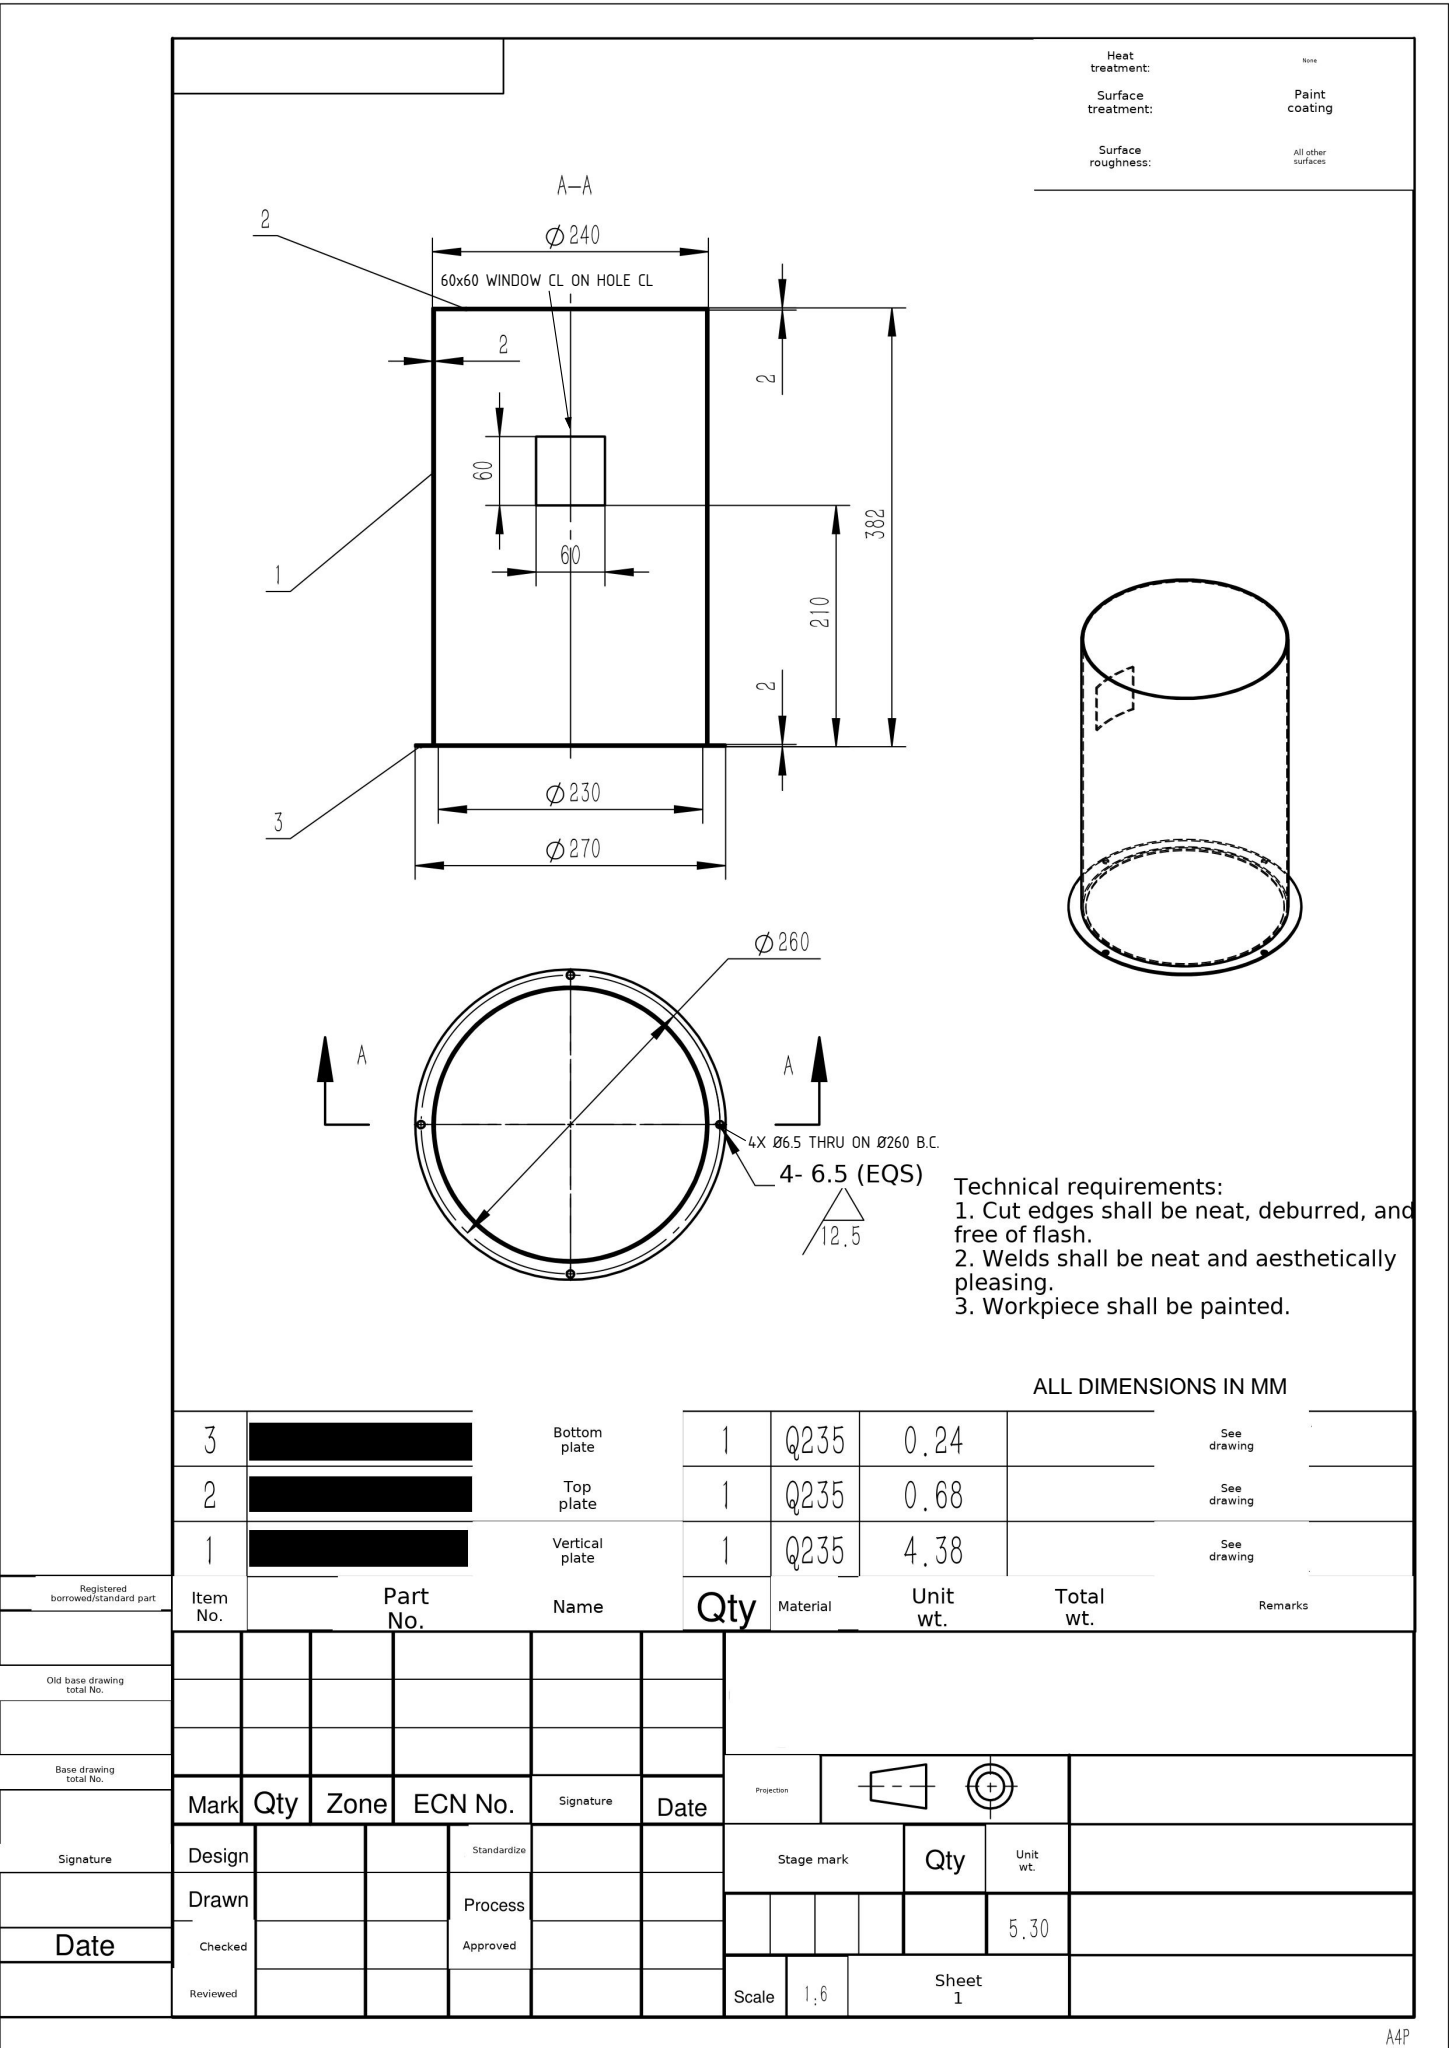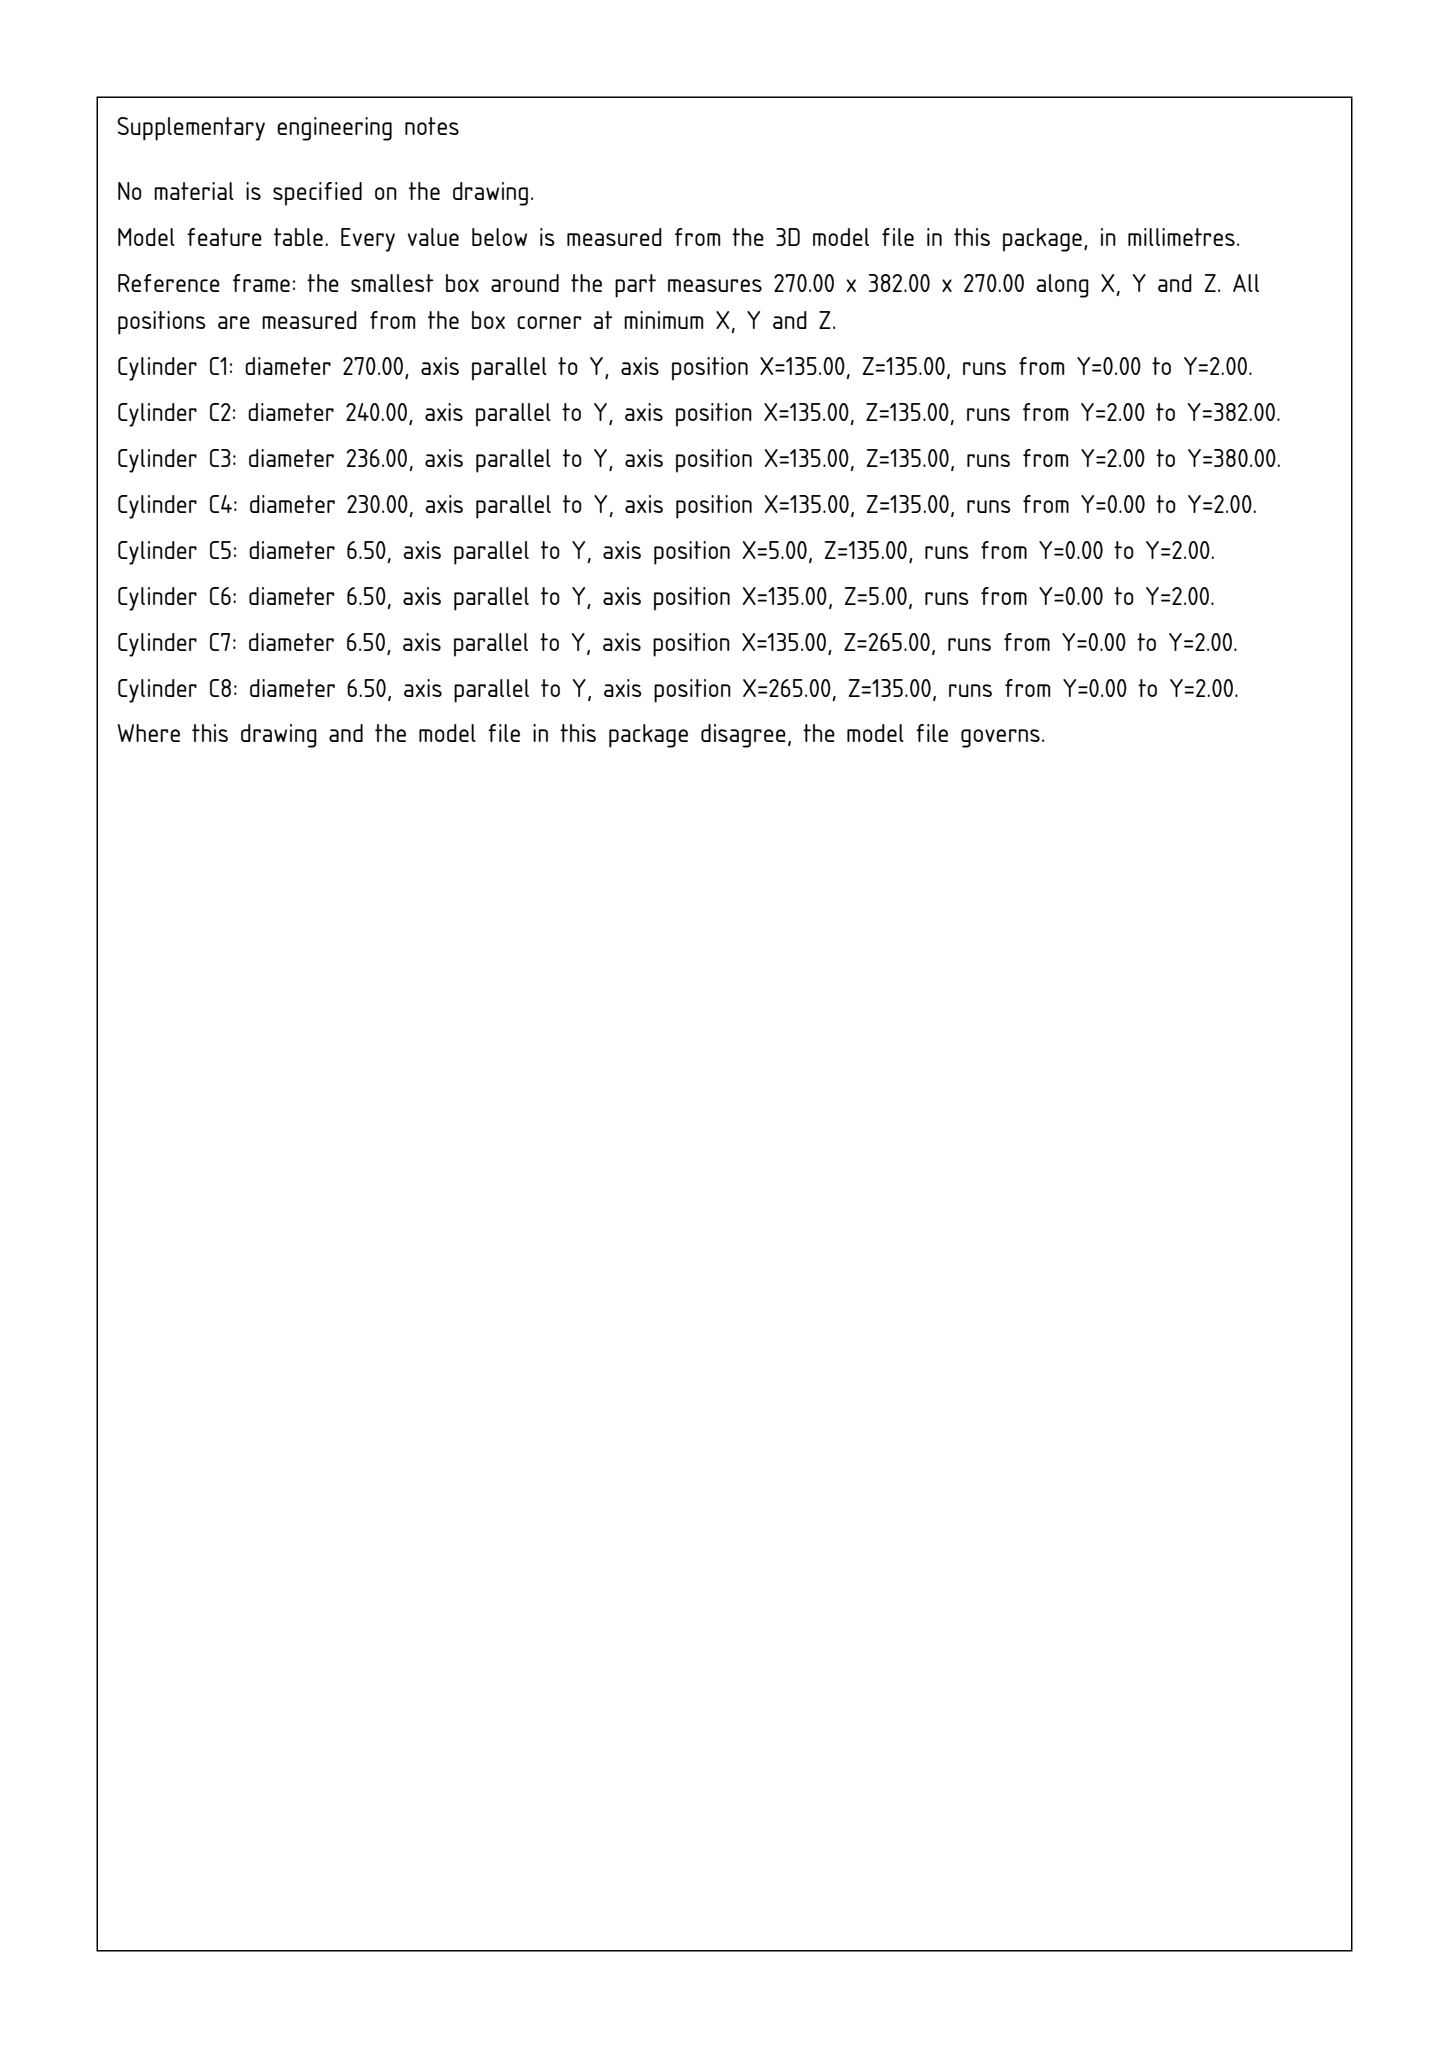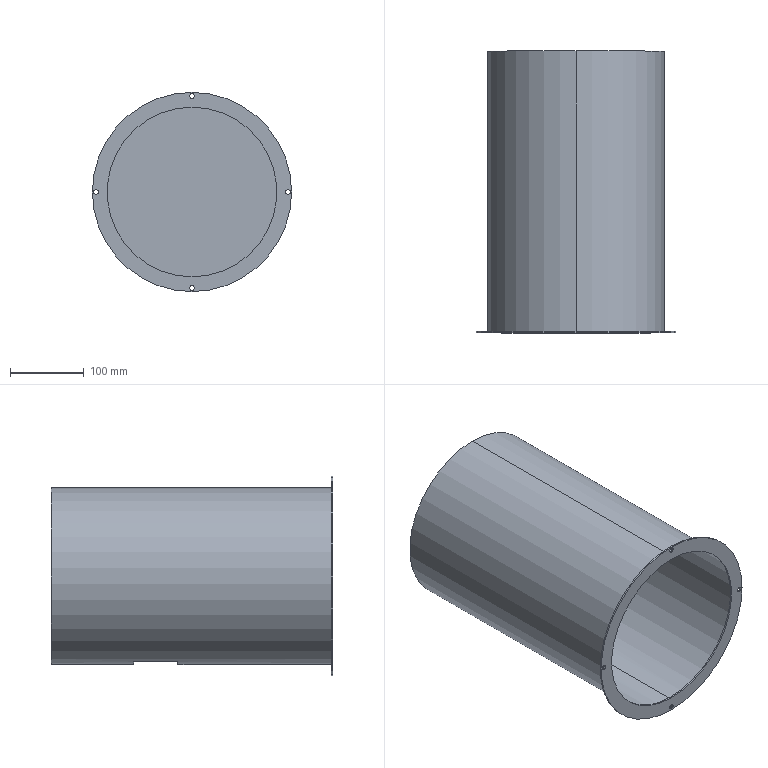Part | SolidWorks | mm | material Q235 | 1 solid | 25 faces | box 270 x 382 x 270 mm | volume 679610 mm3 | cylinder 16 | plane 9 | commonest cylinder face diameters 6.5 x8 230 x2 270 x2 240 x2 236 x2
Drawing notes:
60x60 WINDOW CL ALIGNED W/ ONE 4X Ø6.5 HOLE RADIAL CL (0°) | from the solid: Window faces x=105/165 (CL x=135), z=18.8-20.9; cyl axis at x=135,z=135; Ø6.5 hole at (135,5) lies on same x=135 radial CL
4X Ø6.5 THRU BOTTOM PLATE, EQ SP ON Ø260 B.C. | from the solid: Four Ø6.5 bores, axis y, from y=0 to 2 (2 thk bottom plate), at (135,265),(135,5),(265,135),(5,135) = R130 from axis (135,135)
build123d program:
from build123d import *

# Parameters (mm, degrees)
SKETCH2_R           = 120
SKETCH2_R_2         = 118
BOSS_EXTRUDE1_DEPTH = 380
SKETCH3_R           = 118
BOSS_EXTRUDE2_DEPTH = 2
SKETCH4_R           = 135
SKETCH4_R_2         = 115
BOSS_EXTRUDE3_DEPTH = 2
SKETCH5_R           = 3.25
CUT_EXTRUDE1_DEPTH  = 10
CIRPATTERN1_COUNT   = 4
SKETCH7_W           = 60
SKETCH7_H           = 60
CUT_EXTRUDE5_DEPTH  = 426.265


with BuildPart() as part:
    # Sketch2 → Boss-Extrude1 (new body)
    with BuildSketch(Plane(origin=(0, 0, 0), x_dir=(1, 0, 0), z_dir=(0, 1, 0))):
        with Locations(Location((0, 0, 0), (0, 0, 270))):
            Circle(SKETCH2_R)
        with Locations(Location((0, 0, 0), (0, 0, 270))):
            Circle(SKETCH2_R_2, mode=Mode.SUBTRACT)
    extrude(amount=BOSS_EXTRUDE1_DEPTH)

    # Sketch7 → Cut-Extrude5 (cut, through all)
    with BuildSketch(Plane.XY):
        with Locations((0, 238)):
            Rectangle(SKETCH7_W, SKETCH7_H)
    extrude(amount=-CUT_EXTRUDE5_DEPTH, mode=Mode.SUBTRACT)


with BuildPart() as body_2:
    # Sketch3 → Boss-Extrude2 (new body)
    with BuildSketch(Plane(origin=(0, 380, 0), x_dir=(1, 0, 0), z_dir=(0, 1, 0))):
        with Locations(Location((0, 0, 0), (0, 0, 270))):
            Circle(SKETCH3_R)
    extrude(amount=-BOSS_EXTRUDE2_DEPTH)


with BuildPart() as body_3:
    # Sketch4 → Boss-Extrude3 (new body)
    with BuildSketch(Plane.XZ):
        with Locations(Location((0, 0, 0), (0, 0, 270))):
            Circle(SKETCH4_R)
        with Locations(Location((0, 0, 0), (0, 0, 270))):
            Circle(SKETCH4_R_2, mode=Mode.SUBTRACT)
    extrude(amount=BOSS_EXTRUDE3_DEPTH)

    # Sketch5 → Cut-Extrude1 (cut)
    with BuildSketch(Plane(origin=(0, 0, 0), x_dir=(1, 0, 0), z_dir=(0, 1, 0))):
        with Locations(Location((0, 130, 0), (0, 0, 270))):
            Circle(SKETCH5_R)
    cut_extrude1 = extrude(amount=-CUT_EXTRUDE1_DEPTH, mode=Mode.SUBTRACT)

    # CirPattern1: Cut-Extrude1 ×4 about axis
    cirpattern1_axis = Axis((0, 0, 0), (0, 1, 0))
    for i in range(1, CIRPATTERN1_COUNT):
        add(cut_extrude1.rotate(cirpattern1_axis, i * 360 / CIRPATTERN1_COUNT), mode=Mode.SUBTRACT)


with BuildPart() as part_1:
    add(part.part)

    # Combine-RayDong-Repair: union body 2, body 3
    add(body_2.part)
    add(body_3.part)


solid = part_1.part
STEP:
#1=CARTESIAN_POINT('',(0.,-2.,126.75));
#2=VERTEX_POINT('',#1);
#3=CARTESIAN_POINT('',(-0.,-2.,133.25));
#4=VERTEX_POINT('',#3);
#5=CARTESIAN_POINT('',(0.,-2.,130.));
#6=DIRECTION('',(0.,-1.,0.));
#7=DIRECTION('',(0.,0.,1.));
#8=AXIS2_PLACEMENT_3D('',#5,#6,#7);
#9=CIRCLE('',#8,3.25);
#10=EDGE_CURVE('',#2,#4,#9,.T.);
#11=ORIENTED_EDGE('',*,*,#10,.T.);
#12=CARTESIAN_POINT('',(-0.,0.,133.25));
#13=VERTEX_POINT('',#12);
#14=CARTESIAN_POINT('',(-0.,-10.,133.25));
#15=DIRECTION('',(0.,1.,0.));
#16=VECTOR('',#15,1000.);
#17=LINE('',#14,#16);
#18=EDGE_CURVE('',#4,#13,#17,.T.);
#19=ORIENTED_EDGE('',*,*,#18,.T.);
#20=CARTESIAN_POINT('',(0.,0.,126.75));
#21=VERTEX_POINT('',#20);
#22=CARTESIAN_POINT('',(0.,0.,130.));
#23=DIRECTION('',(0.,1.,0.));
#24=DIRECTION('',(0.,0.,-1.));
#25=AXIS2_PLACEMENT_3D('',#22,#23,#24);
#26=CIRCLE('',#25,3.25);
#27=EDGE_CURVE('',#13,#21,#26,.T.);
#28=ORIENTED_EDGE('',*,*,#27,.T.);
#29=CARTESIAN_POINT('',(0.,-10.,126.75));
#30=DIRECTION('',(0.,1.,0.));
#31=VECTOR('',#30,1000.);
#32=LINE('',#29,#31);
#33=EDGE_CURVE('',#2,#21,#32,.T.);
#34=ORIENTED_EDGE('',*,*,#33,.F.);
#35=EDGE_LOOP('',(#11,#19,#28,#34));
#36=FACE_OUTER_BOUND('',#35,.T.);
#37=CARTESIAN_POINT('',(0.,-10.,130.));
#38=DIRECTION('',(0.,1.,0.));
#39=DIRECTION('',(0.,0.,-1.));
#40=AXIS2_PLACEMENT_3D('',#37,#38,#39);
#41=CYLINDRICAL_SURFACE('',#40,3.25);
#42=ADVANCED_FACE('',(#36),#41,.F.);
#43=CARTESIAN_POINT('',(126.75,-2.,-0.));
#44=VERTEX_POINT('',#43);
#45=CARTESIAN_POINT('',(133.25,-2.,-0.));
#46=VERTEX_POINT('',#45);
#47=CARTESIAN_POINT('',(130.,-2.,-0.));
#48=DIRECTION('',(0.,-1.,0.));
#49=DIRECTION('',(1.,0.,-0.));
#50=AXIS2_PLACEMENT_3D('',#47,#48,#49);
#51=CIRCLE('',#50,3.25);
#52=EDGE_CURVE('',#44,#46,#51,.T.);
#53=ORIENTED_EDGE('',*,*,#52,.T.);
#54=CARTESIAN_POINT('',(133.25,0.,-0.));
#55=VERTEX_POINT('',#54);
#56=CARTESIAN_POINT('',(133.25,-10.,-0.));
#57=DIRECTION('',(0.,1.,0.));
#58=VECTOR('',#57,1000.);
#59=LINE('',#56,#58);
#60=EDGE_CURVE('',#46,#55,#59,.T.);
#61=ORIENTED_EDGE('',*,*,#60,.T.);
#62=CARTESIAN_POINT('',(126.75,0.,-0.));
#63=VERTEX_POINT('',#62);
#64=CARTESIAN_POINT('',(130.,0.,-0.));
#65=DIRECTION('',(0.,1.,0.));
#66=DIRECTION('',(-1.,0.,0.));
#67=AXIS2_PLACEMENT_3D('',#64,#65,#66);
#68=CIRCLE('',#67,3.25);
#69=EDGE_CURVE('',#55,#63,#68,.T.);
#70=ORIENTED_EDGE('',*,*,#69,.T.);
#71=CARTESIAN_POINT('',(126.75,-10.,-0.));
#72=DIRECTION('',(0.,1.,0.));
#73=VECTOR('',#72,1000.);
#74=LINE('',#71,#73);
#75=EDGE_CURVE('',#44,#63,#74,.T.);
#76=ORIENTED_EDGE('',*,*,#75,.F.);
#77=EDGE_LOOP('',(#53,#61,#70,#76));
#78=FACE_OUTER_BOUND('',#77,.T.);
#79=CARTESIAN_POINT('',(130.,-10.,-0.));
#80=DIRECTION('',(0.,1.,0.));
#81=DIRECTION('',(-1.,0.,0.));
#82=AXIS2_PLACEMENT_3D('',#79,#80,#81);
#83=CYLINDRICAL_SURFACE('',#82,3.25);
#84=ADVANCED_FACE('',(#78),#83,.F.);
#85=CARTESIAN_POINT('',(-126.75,-2.,0.));
#86=VERTEX_POINT('',#85);
#87=CARTESIAN_POINT('',(-133.25,-2.,0.));
#88=VERTEX_POINT('',#87);
#89=CARTESIAN_POINT('',(-130.,-2.,0.));
#90=DIRECTION('',(0.,-1.,0.));
#91=DIRECTION('',(-1.,0.,0.));
#92=AXIS2_PLACEMENT_3D('',#89,#90,#91);
#93=CIRCLE('',#92,3.25);
#94=EDGE_CURVE('',#86,#88,#93,.T.);
#95=ORIENTED_EDGE('',*,*,#94,.T.);
#96=CARTESIAN_POINT('',(-133.25,0.,0.));
#97=VERTEX_POINT('',#96);
#98=CARTESIAN_POINT('',(-133.25,-10.,0.));
#99=DIRECTION('',(0.,1.,0.));
#100=VECTOR('',#99,1000.);
#101=LINE('',#98,#100);
#102=EDGE_CURVE('',#88,#97,#101,.T.);
#103=ORIENTED_EDGE('',*,*,#102,.T.);
#104=CARTESIAN_POINT('',(-126.75,0.,0.));
#105=VERTEX_POINT('',#104);
#106=CARTESIAN_POINT('',(-130.,0.,0.));
#107=DIRECTION('',(0.,1.,0.));
#108=DIRECTION('',(1.,0.,-0.));
#109=AXIS2_PLACEMENT_3D('',#106,#107,#108);
#110=CIRCLE('',#109,3.25);
#111=EDGE_CURVE('',#97,#105,#110,.T.);
#112=ORIENTED_EDGE('',*,*,#111,.T.);
#113=CARTESIAN_POINT('',(-126.75,-10.,0.));
#114=DIRECTION('',(0.,1.,0.));
#115=VECTOR('',#114,1000.);
#116=LINE('',#113,#115);
#117=EDGE_CURVE('',#86,#105,#116,.T.);
#118=ORIENTED_EDGE('',*,*,#117,.F.);
#119=EDGE_LOOP('',(#95,#103,#112,#118));
#120=FACE_OUTER_BOUND('',#119,.T.);
#121=CARTESIAN_POINT('',(-130.,-10.,0.));
#122=DIRECTION('',(0.,1.,0.));
#123=DIRECTION('',(1.,0.,-0.));
#124=AXIS2_PLACEMENT_3D('',#121,#122,#123);
#125=CYLINDRICAL_SURFACE('',#124,3.25);
#126=ADVANCED_FACE('',(#120),#125,.F.);
#127=CARTESIAN_POINT('',(0.,-2.,-126.75));
#128=VERTEX_POINT('',#127);
#129=CARTESIAN_POINT('',(0.,-2.,-133.25));
#130=VERTEX_POINT('',#129);
#131=CARTESIAN_POINT('',(0.,-2.,-130.));
#132=DIRECTION('',(0.,-1.,0.));
#133=DIRECTION('',(0.,0.,-1.));
#134=AXIS2_PLACEMENT_3D('',#131,#132,#133);
#135=CIRCLE('',#134,3.25);
#136=EDGE_CURVE('',#128,#130,#135,.T.);
#137=ORIENTED_EDGE('',*,*,#136,.T.);
#138=CARTESIAN_POINT('',(0.,0.,-133.25));
#139=VERTEX_POINT('',#138);
#140=CARTESIAN_POINT('',(0.,-10.,-133.25));
#141=DIRECTION('',(0.,1.,0.));
#142=VECTOR('',#141,1000.);
#143=LINE('',#140,#142);
#144=EDGE_CURVE('',#130,#139,#143,.T.);
#145=ORIENTED_EDGE('',*,*,#144,.T.);
#146=CARTESIAN_POINT('',(0.,0.,-126.75));
#147=VERTEX_POINT('',#146);
#148=CARTESIAN_POINT('',(0.,0.,-130.));
#149=DIRECTION('',(0.,1.,0.));
#150=DIRECTION('',(0.,0.,1.));
#151=AXIS2_PLACEMENT_3D('',#148,#149,#150);
#152=CIRCLE('',#151,3.25);
#153=EDGE_CURVE('',#139,#147,#152,.T.);
#154=ORIENTED_EDGE('',*,*,#153,.T.);
#155=CARTESIAN_POINT('',(0.,-10.,-126.75));
#156=DIRECTION('',(0.,1.,0.));
#157=VECTOR('',#156,1000.);
#158=LINE('',#155,#157);
#159=EDGE_CURVE('',#128,#147,#158,.T.);
#160=ORIENTED_EDGE('',*,*,#159,.F.);
#161=EDGE_LOOP('',(#137,#145,#154,#160));
#162=FACE_OUTER_BOUND('',#161,.T.);
#163=CARTESIAN_POINT('',(0.,-10.,-130.));
#164=DIRECTION('',(0.,1.,0.));
#165=DIRECTION('',(0.,0.,1.));
#166=AXIS2_PLACEMENT_3D('',#163,#164,#165);
#167=CYLINDRICAL_SURFACE('',#166,3.25);
#168=ADVANCED_FACE('',(#162),#167,.F.);
#169=CARTESIAN_POINT('',(0.,-2.,115.));
#170=VERTEX_POINT('',#169);
#171=CARTESIAN_POINT('',(0.,-2.,-115.));
#172=VERTEX_POINT('',#171);
#173=CARTESIAN_POINT('',(0.,-2.,0.));
#174=DIRECTION('',(0.,-1.,0.));
#175=DIRECTION('',(0.,0.,-1.));
#176=AXIS2_PLACEMENT_3D('',#173,#174,#175);
#177=CIRCLE('',#176,115.);
#178=EDGE_CURVE('',#170,#172,#177,.T.);
#179=ORIENTED_EDGE('',*,*,#178,.T.);
#180=CARTESIAN_POINT('',(0.,0.,-115.));
#181=VERTEX_POINT('',#180);
#182=CARTESIAN_POINT('',(0.,-2.,-115.));
#183=DIRECTION('',(0.,1.,0.));
#184=VECTOR('',#183,1000.);
#185=LINE('',#182,#184);
#186=EDGE_CURVE('',#172,#181,#185,.T.);
#187=ORIENTED_EDGE('',*,*,#186,.T.);
#188=CARTESIAN_POINT('',(0.,0.,115.));
#189=VERTEX_POINT('',#188);
#190=CARTESIAN_POINT('',(0.,0.,0.));
#191=DIRECTION('',(0.,-1.,0.));
#192=DIRECTION('',(0.,0.,-1.));
#193=AXIS2_PLACEMENT_3D('',#190,#191,#192);
#194=CIRCLE('',#193,115.);
#195=EDGE_CURVE('',#189,#181,#194,.T.);
#196=ORIENTED_EDGE('',*,*,#195,.F.);
#197=CARTESIAN_POINT('',(0.,-2.,115.));
#198=DIRECTION('',(0.,1.,0.));
#199=VECTOR('',#198,1000.);
#200=LINE('',#197,#199);
#201=EDGE_CURVE('',#170,#189,#200,.T.);
#202=ORIENTED_EDGE('',*,*,#201,.F.);
#203=EDGE_LOOP('',(#179,#187,#196,#202));
#204=FACE_OUTER_BOUND('',#203,.T.);
#205=CARTESIAN_POINT('',(0.,-2.,0.));
#206=DIRECTION('',(0.,1.,0.));
#207=DIRECTION('',(0.,0.,1.));
#208=AXIS2_PLACEMENT_3D('',#205,#206,#207);
#209=CYLINDRICAL_SURFACE('',#208,115.);
#210=ADVANCED_FACE('',(#204),#209,.F.);
#211=CARTESIAN_POINT('',(0.,-2.,-135.));
#212=VERTEX_POINT('',#211);
#213=CARTESIAN_POINT('',(0.,-2.,135.));
#214=VERTEX_POINT('',#213);
#215=CARTESIAN_POINT('',(0.,-2.,0.));
#216=DIRECTION('',(0.,-1.,0.));
#217=DIRECTION('',(0.,0.,-1.));
#218=AXIS2_PLACEMENT_3D('',#215,#216,#217);
#219=CIRCLE('',#218,135.);
#220=EDGE_CURVE('',#212,#214,#219,.T.);
#221=ORIENTED_EDGE('',*,*,#220,.F.);
#222=CARTESIAN_POINT('',(0.,0.,-135.));
#223=VERTEX_POINT('',#222);
#224=CARTESIAN_POINT('',(0.,-2.,-135.));
#225=DIRECTION('',(0.,1.,0.));
#226=VECTOR('',#225,1000.);
#227=LINE('',#224,#226);
#228=EDGE_CURVE('',#212,#223,#227,.T.);
#229=ORIENTED_EDGE('',*,*,#228,.T.);
#230=CARTESIAN_POINT('',(0.,0.,135.));
#231=VERTEX_POINT('',#230);
#232=CARTESIAN_POINT('',(0.,0.,0.));
#233=DIRECTION('',(0.,-1.,0.));
#234=DIRECTION('',(0.,0.,-1.));
#235=AXIS2_PLACEMENT_3D('',#232,#233,#234);
#236=CIRCLE('',#235,135.);
#237=EDGE_CURVE('',#223,#231,#236,.T.);
#238=ORIENTED_EDGE('',*,*,#237,.T.);
#239=CARTESIAN_POINT('',(0.,-2.,135.));
#240=DIRECTION('',(0.,1.,0.));
#241=VECTOR('',#240,1000.);
#242=LINE('',#239,#241);
#243=EDGE_CURVE('',#214,#231,#242,.T.);
#244=ORIENTED_EDGE('',*,*,#243,.F.);
#245=EDGE_LOOP('',(#221,#229,#238,#244));
#246=FACE_OUTER_BOUND('',#245,.T.);
#247=CARTESIAN_POINT('',(0.,-2.,0.));
#248=DIRECTION('',(0.,1.,0.));
#249=DIRECTION('',(0.,0.,1.));
#250=AXIS2_PLACEMENT_3D('',#247,#248,#249);
#251=CYLINDRICAL_SURFACE('',#250,135.);
#252=ADVANCED_FACE('',(#246),#251,.T.);
#253=CARTESIAN_POINT('',(0.,380.,120.));
#254=VERTEX_POINT('',#253);
#255=CARTESIAN_POINT('',(0.,380.,-120.));
#256=VERTEX_POINT('',#255);
#257=CARTESIAN_POINT('',(0.,380.,0.));
#258=DIRECTION('',(0.,1.,0.));
#259=DIRECTION('',(0.,0.,1.));
#260=AXIS2_PLACEMENT_3D('',#257,#258,#259);
#261=CIRCLE('',#260,120.);
#262=EDGE_CURVE('',#254,#256,#261,.T.);
#263=ORIENTED_EDGE('',*,*,#262,.F.);
#264=CARTESIAN_POINT('',(0.,0.,120.));
#265=VERTEX_POINT('',#264);
#266=CARTESIAN_POINT('',(0.,380.,120.));
#267=DIRECTION('',(0.,-1.,0.));
#268=VECTOR('',#267,1000.);
#269=LINE('',#266,#268);
#270=EDGE_CURVE('',#254,#265,#269,.T.);
#271=ORIENTED_EDGE('',*,*,#270,.T.);
#272=CARTESIAN_POINT('',(0.,0.,-120.));
#273=VERTEX_POINT('',#272);
#274=CARTESIAN_POINT('',(0.,0.,0.));
#275=DIRECTION('',(0.,1.,0.));
#276=DIRECTION('',(0.,0.,1.));
#277=AXIS2_PLACEMENT_3D('',#274,#275,#276);
#278=CIRCLE('',#277,120.);
#279=EDGE_CURVE('',#265,#273,#278,.T.);
#280=ORIENTED_EDGE('',*,*,#279,.T.);
#281=CARTESIAN_POINT('',(0.,208.,-120.));
#282=VERTEX_POINT('',#281);
#283=CARTESIAN_POINT('',(0.,380.,-120.));
#284=DIRECTION('',(0.,-1.,0.));
#285=VECTOR('',#284,1000.);
#286=LINE('',#283,#285);
#287=EDGE_CURVE('',#282,#273,#286,.T.);
#288=ORIENTED_EDGE('',*,*,#287,.F.);
#289=CARTESIAN_POINT('',(30.,208.,-116.19));
#290=VERTEX_POINT('',#289);
#291=CARTESIAN_POINT('',(0.,208.,0.));
#292=DIRECTION('',(0.,-1.,0.));
#293=DIRECTION('',(0.,0.,-1.));
#294=AXIS2_PLACEMENT_3D('',#291,#292,#293);
#295=CIRCLE('',#294,120.);
#296=EDGE_CURVE('',#282,#290,#295,.T.);
#297=ORIENTED_EDGE('',*,*,#296,.T.);
#298=CARTESIAN_POINT('',(30.,268.,-116.19));
#299=VERTEX_POINT('',#298);
#300=CARTESIAN_POINT('',(30.,380.,-116.19));
#301=DIRECTION('',(0.,1.,0.));
#302=VECTOR('',#301,1000.);
#303=LINE('',#300,#302);
#304=EDGE_CURVE('',#290,#299,#303,.T.);
#305=ORIENTED_EDGE('',*,*,#304,.T.);
#306=CARTESIAN_POINT('',(0.,268.,-120.));
#307=VERTEX_POINT('',#306);
#308=CARTESIAN_POINT('',(0.,268.,0.));
#309=DIRECTION('',(0.,1.,0.));
#310=DIRECTION('',(0.,0.,1.));
#311=AXIS2_PLACEMENT_3D('',#308,#309,#310);
#312=CIRCLE('',#311,120.);
#313=EDGE_CURVE('',#299,#307,#312,.T.);
#314=ORIENTED_EDGE('',*,*,#313,.T.);
#315=CARTESIAN_POINT('',(0.,380.,-120.));
#316=DIRECTION('',(0.,-1.,0.));
#317=VECTOR('',#316,1000.);
#318=LINE('',#315,#317);
#319=EDGE_CURVE('',#256,#307,#318,.T.);
#320=ORIENTED_EDGE('',*,*,#319,.F.);
#321=EDGE_LOOP('',(#263,#271,#280,#288,#297,#305,#314,#320));
#322=FACE_OUTER_BOUND('',#321,.T.);
#323=CARTESIAN_POINT('',(0.,380.,0.));
#324=DIRECTION('',(0.,-1.,0.));
#325=DIRECTION('',(0.,0.,-1.));
#326=AXIS2_PLACEMENT_3D('',#323,#324,#325);
#327=CYLINDRICAL_SURFACE('',#326,120.);
#328=ADVANCED_FACE('',(#322),#327,.T.);
#329=CARTESIAN_POINT('',(0.,378.,-118.));
#330=VERTEX_POINT('',#329);
#331=CARTESIAN_POINT('',(0.,378.,118.));
#332=VERTEX_POINT('',#331);
#333=CARTESIAN_POINT('',(0.,378.,0.));
#334=DIRECTION('',(0.,1.,0.));
#335=DIRECTION('',(0.,0.,1.));
#336=AXIS2_PLACEMENT_3D('',#333,#334,#335);
#337=CIRCLE('',#336,118.);
#338=EDGE_CURVE('',#330,#332,#337,.T.);
#339=ORIENTED_EDGE('',*,*,#338,.T.);
#340=CARTESIAN_POINT('',(0.,0.,118.));
#341=VERTEX_POINT('',#340);
#342=CARTESIAN_POINT('',(0.,380.,118.));
#343=DIRECTION('',(0.,-1.,0.));
#344=VECTOR('',#343,1000.);
#345=LINE('',#342,#344);
#346=EDGE_CURVE('',#332,#341,#345,.T.);
#347=ORIENTED_EDGE('',*,*,#346,.T.);
#348=CARTESIAN_POINT('',(0.,0.,-118.));
#349=VERTEX_POINT('',#348);
#350=CARTESIAN_POINT('',(0.,0.,0.));
#351=DIRECTION('',(0.,1.,0.));
#352=DIRECTION('',(0.,0.,1.));
#353=AXIS2_PLACEMENT_3D('',#350,#351,#352);
#354=CIRCLE('',#353,118.);
#355=EDGE_CURVE('',#349,#341,#354,.T.);
#356=ORIENTED_EDGE('',*,*,#355,.F.);
#357=CARTESIAN_POINT('',(0.,208.,-118.));
#358=VERTEX_POINT('',#357);
#359=CARTESIAN_POINT('',(0.,380.,-118.));
#360=DIRECTION('',(0.,-1.,0.));
#361=VECTOR('',#360,1000.);
#362=LINE('',#359,#361);
#363=EDGE_CURVE('',#358,#349,#362,.T.);
#364=ORIENTED_EDGE('',*,*,#363,.F.);
#365=CARTESIAN_POINT('',(-30.,208.,-114.123));
#366=VERTEX_POINT('',#365);
#367=CARTESIAN_POINT('',(0.,208.,0.));
#368=DIRECTION('',(0.,-1.,0.));
#369=DIRECTION('',(0.,0.,-1.));
#370=AXIS2_PLACEMENT_3D('',#367,#368,#369);
#371=CIRCLE('',#370,118.);
#372=EDGE_CURVE('',#366,#358,#371,.T.);
#373=ORIENTED_EDGE('',*,*,#372,.F.);
#374=CARTESIAN_POINT('',(-30.,268.,-114.123));
#375=VERTEX_POINT('',#374);
#376=CARTESIAN_POINT('',(-30.,380.,-114.123));
#377=DIRECTION('',(0.,-1.,0.));
#378=VECTOR('',#377,1000.);
#379=LINE('',#376,#378);
#380=EDGE_CURVE('',#375,#366,#379,.T.);
#381=ORIENTED_EDGE('',*,*,#380,.F.);
#382=CARTESIAN_POINT('',(0.,268.,-118.));
#383=VERTEX_POINT('',#382);
#384=CARTESIAN_POINT('',(0.,268.,0.));
#385=DIRECTION('',(0.,1.,0.));
#386=DIRECTION('',(0.,0.,1.));
#387=AXIS2_PLACEMENT_3D('',#384,#385,#386);
#388=CIRCLE('',#387,118.);
#389=EDGE_CURVE('',#383,#375,#388,.T.);
#390=ORIENTED_EDGE('',*,*,#389,.F.);
#391=CARTESIAN_POINT('',(0.,380.,-118.));
#392=DIRECTION('',(0.,-1.,0.));
#393=VECTOR('',#392,1000.);
#394=LINE('',#391,#393);
#395=EDGE_CURVE('',#330,#383,#394,.T.);
#396=ORIENTED_EDGE('',*,*,#395,.F.);
#397=EDGE_LOOP('',(#339,#347,#356,#364,#373,#381,#390,#396));
#398=FACE_OUTER_BOUND('',#397,.T.);
#399=CARTESIAN_POINT('',(0.,380.,0.));
#400=DIRECTION('',(0.,-1.,0.));
#401=DIRECTION('',(0.,0.,-1.));
#402=AXIS2_PLACEMENT_3D('',#399,#400,#401);
#403=CYLINDRICAL_SURFACE('',#402,118.);
#404=ADVANCED_FACE('',(#398),#403,.F.);
#405=ORIENTED_EDGE('',*,*,#346,.F.);
#406=CARTESIAN_POINT('',(0.,378.,0.));
#407=DIRECTION('',(0.,1.,0.));
#408=DIRECTION('',(0.,0.,1.));
#409=AXIS2_PLACEMENT_3D('',#406,#407,#408);
#410=CIRCLE('',#409,118.);
#411=EDGE_CURVE('',#332,#330,#410,.T.);
#412=ORIENTED_EDGE('',*,*,#411,.T.);
#413=ORIENTED_EDGE('',*,*,#395,.T.);
#414=CARTESIAN_POINT('',(30.,268.,-114.123));
#415=VERTEX_POINT('',#414);
#416=CARTESIAN_POINT('',(0.,268.,0.));
#417=DIRECTION('',(0.,1.,0.));
#418=DIRECTION('',(0.,0.,1.));
#419=AXIS2_PLACEMENT_3D('',#416,#417,#418);
#420=CIRCLE('',#419,118.);
#421=EDGE_CURVE('',#415,#383,#420,.T.);
#422=ORIENTED_EDGE('',*,*,#421,.F.);
#423=CARTESIAN_POINT('',(30.,208.,-114.123));
#424=VERTEX_POINT('',#423);
#425=CARTESIAN_POINT('',(30.,380.,-114.123));
#426=DIRECTION('',(0.,1.,0.));
#427=VECTOR('',#426,1000.);
#428=LINE('',#425,#427);
#429=EDGE_CURVE('',#424,#415,#428,.T.);
#430=ORIENTED_EDGE('',*,*,#429,.F.);
#431=CARTESIAN_POINT('',(0.,208.,0.));
#432=DIRECTION('',(0.,-1.,0.));
#433=DIRECTION('',(0.,0.,-1.));
#434=AXIS2_PLACEMENT_3D('',#431,#432,#433);
#435=CIRCLE('',#434,118.);
#436=EDGE_CURVE('',#358,#424,#435,.T.);
#437=ORIENTED_EDGE('',*,*,#436,.F.);
#438=ORIENTED_EDGE('',*,*,#363,.T.);
#439=CARTESIAN_POINT('',(0.,0.,0.));
#440=DIRECTION('',(0.,1.,0.));
#441=DIRECTION('',(0.,0.,1.));
#442=AXIS2_PLACEMENT_3D('',#439,#440,#441);
#443=CIRCLE('',#442,118.);
#444=EDGE_CURVE('',#341,#349,#443,.T.);
#445=ORIENTED_EDGE('',*,*,#444,.F.);
#446=EDGE_LOOP('',(#405,#412,#413,#422,#430,#437,#438,#445));
#447=FACE_OUTER_BOUND('',#446,.T.);
#448=CARTESIAN_POINT('',(0.,380.,0.));
#449=DIRECTION('',(0.,-1.,0.));
#450=DIRECTION('',(0.,0.,-1.));
#451=AXIS2_PLACEMENT_3D('',#448,#449,#450);
#452=CYLINDRICAL_SURFACE('',#451,118.);
#453=ADVANCED_FACE('',(#447),#452,.F.);
#454=CARTESIAN_POINT('',(0.,380.,0.));
#455=DIRECTION('',(0.,1.,0.));
#456=DIRECTION('',(0.,0.,1.));
#457=AXIS2_PLACEMENT_3D('',#454,#455,#456);
#458=CIRCLE('',#457,120.);
#459=EDGE_CURVE('',#256,#254,#458,.T.);
#460=ORIENTED_EDGE('',*,*,#459,.T.);
#461=ORIENTED_EDGE('',*,*,#262,.T.);
#462=EDGE_LOOP('',(#460,#461));
#463=FACE_OUTER_BOUND('',#462,.T.);
#464=CARTESIAN_POINT('',(0.,380.,0.));
#465=DIRECTION('',(0.,1.,0.));
#466=DIRECTION('',(0.,0.,1.));
#467=AXIS2_PLACEMENT_3D('',#464,#465,#466);
#468=PLANE('',#467);
#469=ADVANCED_FACE('',(#463),#468,.T.);
#470=ORIENTED_EDGE('',*,*,#270,.F.);
#471=ORIENTED_EDGE('',*,*,#459,.F.);
#472=ORIENTED_EDGE('',*,*,#319,.T.);
#473=CARTESIAN_POINT('',(-30.,268.,-116.19));
#474=VERTEX_POINT('',#473);
#475=CARTESIAN_POINT('',(0.,268.,0.));
#476=DIRECTION('',(0.,1.,0.));
#477=DIRECTION('',(0.,0.,1.));
#478=AXIS2_PLACEMENT_3D('',#475,#476,#477);
#479=CIRCLE('',#478,120.);
#480=EDGE_CURVE('',#307,#474,#479,.T.);
#481=ORIENTED_EDGE('',*,*,#480,.T.);
#482=CARTESIAN_POINT('',(-30.,208.,-116.19));
#483=VERTEX_POINT('',#482);
#484=CARTESIAN_POINT('',(-30.,380.,-116.19));
#485=DIRECTION('',(0.,-1.,0.));
#486=VECTOR('',#485,1000.);
#487=LINE('',#484,#486);
#488=EDGE_CURVE('',#474,#483,#487,.T.);
#489=ORIENTED_EDGE('',*,*,#488,.T.);
#490=CARTESIAN_POINT('',(0.,208.,0.));
#491=DIRECTION('',(0.,-1.,0.));
#492=DIRECTION('',(0.,0.,-1.));
#493=AXIS2_PLACEMENT_3D('',#490,#491,#492);
#494=CIRCLE('',#493,120.);
#495=EDGE_CURVE('',#483,#282,#494,.T.);
#496=ORIENTED_EDGE('',*,*,#495,.T.);
#497=ORIENTED_EDGE('',*,*,#287,.T.);
#498=CARTESIAN_POINT('',(0.,0.,0.));
#499=DIRECTION('',(0.,1.,0.));
#500=DIRECTION('',(0.,0.,1.));
#501=AXIS2_PLACEMENT_3D('',#498,#499,#500);
#502=CIRCLE('',#501,120.);
#503=EDGE_CURVE('',#273,#265,#502,.T.);
#504=ORIENTED_EDGE('',*,*,#503,.T.);
#505=EDGE_LOOP('',(#470,#471,#472,#481,#489,#496,#497,#504));
#506=FACE_OUTER_BOUND('',#505,.T.);
#507=CARTESIAN_POINT('',(0.,380.,0.));
#508=DIRECTION('',(0.,-1.,0.));
#509=DIRECTION('',(0.,0.,-1.));
#510=AXIS2_PLACEMENT_3D('',#507,#508,#509);
#511=CYLINDRICAL_SURFACE('',#510,120.);
#512=ADVANCED_FACE('',(#506),#511,.T.);
#513=CARTESIAN_POINT('',(30.,208.,-135.));
#514=DIRECTION('',(0.,0.,1.));
#515=VECTOR('',#514,1000.);
#516=LINE('',#513,#515);
#517=EDGE_CURVE('',#290,#424,#516,.T.);
#518=ORIENTED_EDGE('',*,*,#517,.T.);
#519=ORIENTED_EDGE('',*,*,#429,.T.);
#520=CARTESIAN_POINT('',(30.,268.,-135.));
#521=DIRECTION('',(0.,0.,1.));
#522=VECTOR('',#521,1000.);
#523=LINE('',#520,#522);
#524=EDGE_CURVE('',#299,#415,#523,.T.);
#525=ORIENTED_EDGE('',*,*,#524,.F.);
#526=ORIENTED_EDGE('',*,*,#304,.F.);
#527=EDGE_LOOP('',(#518,#519,#525,#526));
#528=FACE_OUTER_BOUND('',#527,.T.);
#529=CARTESIAN_POINT('',(30.,268.,-135.));
#530=DIRECTION('',(1.,0.,0.));
#531=DIRECTION('',(-0.,1.,0.));
#532=AXIS2_PLACEMENT_3D('',#529,#530,#531);
#533=PLANE('',#532);
#534=ADVANCED_FACE('',(#528),#533,.F.);
#535=CARTESIAN_POINT('',(-30.,208.,-135.));
#536=DIRECTION('',(0.,0.,1.));
#537=VECTOR('',#536,1000.);
#538=LINE('',#535,#537);
#539=EDGE_CURVE('',#483,#366,#538,.T.);
#540=ORIENTED_EDGE('',*,*,#539,.T.);
#541=ORIENTED_EDGE('',*,*,#372,.T.);
#542=ORIENTED_EDGE('',*,*,#436,.T.);
#543=ORIENTED_EDGE('',*,*,#517,.F.);
#544=ORIENTED_EDGE('',*,*,#296,.F.);
#545=ORIENTED_EDGE('',*,*,#495,.F.);
#546=EDGE_LOOP('',(#540,#541,#542,#543,#544,#545));
#547=FACE_OUTER_BOUND('',#546,.T.);
#548=CARTESIAN_POINT('',(-30.,208.,-135.));
#549=DIRECTION('',(0.,-1.,0.));
#550=DIRECTION('',(0.,0.,-1.));
#551=AXIS2_PLACEMENT_3D('',#548,#549,#550);
#552=PLANE('',#551);
#553=ADVANCED_FACE('',(#547),#552,.F.);
#554=CARTESIAN_POINT('',(-30.,268.,-135.));
#555=DIRECTION('',(0.,0.,1.));
#556=VECTOR('',#555,1000.);
#557=LINE('',#554,#556);
#558=EDGE_CURVE('',#474,#375,#557,.T.);
#559=ORIENTED_EDGE('',*,*,#558,.T.);
#560=ORIENTED_EDGE('',*,*,#380,.T.);
#561=ORIENTED_EDGE('',*,*,#539,.F.);
#562=ORIENTED_EDGE('',*,*,#488,.F.);
#563=EDGE_LOOP('',(#559,#560,#561,#562));
#564=FACE_OUTER_BOUND('',#563,.T.);
#565=CARTESIAN_POINT('',(-30.,268.,-135.));
#566=DIRECTION('',(-1.,-0.,0.));
#567=DIRECTION('',(0.,-1.,0.));
#568=AXIS2_PLACEMENT_3D('',#565,#566,#567);
#569=PLANE('',#568);
#570=ADVANCED_FACE('',(#564),#569,.F.);
#571=ORIENTED_EDGE('',*,*,#524,.T.);
#572=ORIENTED_EDGE('',*,*,#421,.T.);
#573=ORIENTED_EDGE('',*,*,#389,.T.);
#574=ORIENTED_EDGE('',*,*,#558,.F.);
#575=ORIENTED_EDGE('',*,*,#480,.F.);
#576=ORIENTED_EDGE('',*,*,#313,.F.);
#577=EDGE_LOOP('',(#571,#572,#573,#574,#575,#576));
#578=FACE_OUTER_BOUND('',#577,.T.);
#579=CARTESIAN_POINT('',(-30.,268.,-135.));
#580=DIRECTION('',(0.,1.,0.));
#581=DIRECTION('',(0.,0.,1.));
#582=AXIS2_PLACEMENT_3D('',#579,#580,#581);
#583=PLANE('',#582);
#584=ADVANCED_FACE('',(#578),#583,.F.);
#585=ORIENTED_EDGE('',*,*,#338,.F.);
#586=ORIENTED_EDGE('',*,*,#411,.F.);
#587=EDGE_LOOP('',(#585,#586));
#588=FACE_OUTER_BOUND('',#587,.T.);
#589=CARTESIAN_POINT('',(0.,378.,0.));
#590=DIRECTION('',(0.,1.,0.));
#591=DIRECTION('',(0.,0.,1.));
#592=AXIS2_PLACEMENT_3D('',#589,#590,#591);
#593=PLANE('',#592);
#594=ADVANCED_FACE('',(#588),#593,.F.);
#595=ORIENTED_EDGE('',*,*,#195,.T.);
#596=CARTESIAN_POINT('',(0.,0.,0.));
#597=DIRECTION('',(0.,-1.,0.));
#598=DIRECTION('',(0.,0.,-1.));
#599=AXIS2_PLACEMENT_3D('',#596,#597,#598);
#600=CIRCLE('',#599,115.);
#601=EDGE_CURVE('',#181,#189,#600,.T.);
#602=ORIENTED_EDGE('',*,*,#601,.T.);
#603=EDGE_LOOP('',(#595,#602));
#604=FACE_BOUND('',#603,.T.);
#605=ORIENTED_EDGE('',*,*,#355,.T.);
#606=ORIENTED_EDGE('',*,*,#444,.T.);
#607=EDGE_LOOP('',(#605,#606));
#608=FACE_OUTER_BOUND('',#607,.T.);
#609=CARTESIAN_POINT('',(0.,0.,0.));
#610=DIRECTION('',(0.,-1.,0.));
#611=DIRECTION('',(0.,0.,-1.));
#612=AXIS2_PLACEMENT_3D('',#609,#610,#611);
#613=PLANE('',#612);
#614=ADVANCED_FACE('',(#604,#608),#613,.F.);
#615=ORIENTED_EDGE('',*,*,#10,.F.);
#616=CARTESIAN_POINT('',(0.,-2.,130.));
#617=DIRECTION('',(0.,-1.,0.));
#618=DIRECTION('',(0.,0.,1.));
#619=AXIS2_PLACEMENT_3D('',#616,#617,#618);
#620=CIRCLE('',#619,3.25);
#621=EDGE_CURVE('',#4,#2,#620,.T.);
#622=ORIENTED_EDGE('',*,*,#621,.F.);
#623=EDGE_LOOP('',(#615,#622));
#624=FACE_BOUND('',#623,.T.);
#625=ORIENTED_EDGE('',*,*,#52,.F.);
#626=CARTESIAN_POINT('',(130.,-2.,-0.));
#627=DIRECTION('',(0.,-1.,0.));
#628=DIRECTION('',(1.,0.,-0.));
#629=AXIS2_PLACEMENT_3D('',#626,#627,#628);
#630=CIRCLE('',#629,3.25);
#631=EDGE_CURVE('',#46,#44,#630,.T.);
#632=ORIENTED_EDGE('',*,*,#631,.F.);
#633=EDGE_LOOP('',(#625,#632));
#634=FACE_BOUND('',#633,.T.);
#635=ORIENTED_EDGE('',*,*,#94,.F.);
#636=CARTESIAN_POINT('',(-130.,-2.,0.));
#637=DIRECTION('',(0.,-1.,0.));
#638=DIRECTION('',(-1.,0.,0.));
#639=AXIS2_PLACEMENT_3D('',#636,#637,#638);
#640=CIRCLE('',#639,3.25);
#641=EDGE_CURVE('',#88,#86,#640,.T.);
#642=ORIENTED_EDGE('',*,*,#641,.F.);
#643=EDGE_LOOP('',(#635,#642));
#644=FACE_BOUND('',#643,.T.);
#645=ORIENTED_EDGE('',*,*,#136,.F.);
#646=CARTESIAN_POINT('',(0.,-2.,-130.));
#647=DIRECTION('',(0.,-1.,0.));
#648=DIRECTION('',(0.,0.,-1.));
#649=AXIS2_PLACEMENT_3D('',#646,#647,#648);
#650=CIRCLE('',#649,3.25);
#651=EDGE_CURVE('',#130,#128,#650,.T.);
#652=ORIENTED_EDGE('',*,*,#651,.F.);
#653=EDGE_LOOP('',(#645,#652));
#654=FACE_BOUND('',#653,.T.);
#655=CARTESIAN_POINT('',(0.,-2.,0.));
#656=DIRECTION('',(0.,-1.,0.));
#657=DIRECTION('',(0.,0.,-1.));
#658=AXIS2_PLACEMENT_3D('',#655,#656,#657);
#659=CIRCLE('',#658,135.);
#660=EDGE_CURVE('',#214,#212,#659,.T.);
#661=ORIENTED_EDGE('',*,*,#660,.T.);
#662=ORIENTED_EDGE('',*,*,#220,.T.);
#663=EDGE_LOOP('',(#661,#662));
#664=FACE_OUTER_BOUND('',#663,.T.);
#665=ORIENTED_EDGE('',*,*,#178,.F.);
#666=CARTESIAN_POINT('',(0.,-2.,0.));
#667=DIRECTION('',(0.,-1.,0.));
#668=DIRECTION('',(0.,0.,-1.));
#669=AXIS2_PLACEMENT_3D('',#666,#667,#668);
#670=CIRCLE('',#669,115.);
#671=EDGE_CURVE('',#172,#170,#670,.T.);
#672=ORIENTED_EDGE('',*,*,#671,.F.);
#673=EDGE_LOOP('',(#665,#672));
#674=FACE_BOUND('',#673,.T.);
#675=CARTESIAN_POINT('',(0.,-2.,0.));
#676=DIRECTION('',(0.,-1.,0.));
#677=DIRECTION('',(0.,0.,-1.));
#678=AXIS2_PLACEMENT_3D('',#675,#676,#677);
#679=PLANE('',#678);
#680=ADVANCED_FACE('',(#624,#634,#644,#654,#664,#674),#679,.T.);
#681=ORIENTED_EDGE('',*,*,#503,.F.);
#682=ORIENTED_EDGE('',*,*,#279,.F.);
#683=EDGE_LOOP('',(#681,#682));
#684=FACE_BOUND('',#683,.T.);
#685=CARTESIAN_POINT('',(0.,0.,130.));
#686=DIRECTION('',(0.,1.,0.));
#687=DIRECTION('',(0.,0.,-1.));
#688=AXIS2_PLACEMENT_3D('',#685,#686,#687);
#689=CIRCLE('',#688,3.25);
#690=EDGE_CURVE('',#21,#13,#689,.T.);
#691=ORIENTED_EDGE('',*,*,#690,.F.);
#692=ORIENTED_EDGE('',*,*,#27,.F.);
#693=EDGE_LOOP('',(#691,#692));
#694=FACE_BOUND('',#693,.T.);
#695=CARTESIAN_POINT('',(130.,0.,-0.));
#696=DIRECTION('',(0.,1.,0.));
#697=DIRECTION('',(-1.,0.,0.));
#698=AXIS2_PLACEMENT_3D('',#695,#696,#697);
#699=CIRCLE('',#698,3.25);
#700=EDGE_CURVE('',#63,#55,#699,.T.);
#701=ORIENTED_EDGE('',*,*,#700,.F.);
#702=ORIENTED_EDGE('',*,*,#69,.F.);
#703=EDGE_LOOP('',(#701,#702));
#704=FACE_BOUND('',#703,.T.);
#705=CARTESIAN_POINT('',(-130.,0.,0.));
#706=DIRECTION('',(0.,1.,0.));
#707=DIRECTION('',(1.,0.,-0.));
#708=AXIS2_PLACEMENT_3D('',#705,#706,#707);
#709=CIRCLE('',#708,3.25);
#710=EDGE_CURVE('',#105,#97,#709,.T.);
#711=ORIENTED_EDGE('',*,*,#710,.F.);
#712=ORIENTED_EDGE('',*,*,#111,.F.);
#713=EDGE_LOOP('',(#711,#712));
#714=FACE_BOUND('',#713,.T.);
#715=CARTESIAN_POINT('',(0.,0.,-130.));
#716=DIRECTION('',(0.,1.,0.));
#717=DIRECTION('',(0.,0.,1.));
#718=AXIS2_PLACEMENT_3D('',#715,#716,#717);
#719=CIRCLE('',#718,3.25);
#720=EDGE_CURVE('',#147,#139,#719,.T.);
#721=ORIENTED_EDGE('',*,*,#720,.F.);
#722=ORIENTED_EDGE('',*,*,#153,.F.);
#723=EDGE_LOOP('',(#721,#722));
#724=FACE_BOUND('',#723,.T.);
#725=CARTESIAN_POINT('',(0.,0.,0.));
#726=DIRECTION('',(0.,-1.,0.));
#727=DIRECTION('',(0.,0.,-1.));
#728=AXIS2_PLACEMENT_3D('',#725,#726,#727);
#729=CIRCLE('',#728,135.);
#730=EDGE_CURVE('',#231,#223,#729,.T.);
#731=ORIENTED_EDGE('',*,*,#730,.F.);
#732=ORIENTED_EDGE('',*,*,#237,.F.);
#733=EDGE_LOOP('',(#731,#732));
#734=FACE_OUTER_BOUND('',#733,.T.);
#735=CARTESIAN_POINT('',(0.,0.,0.));
#736=DIRECTION('',(0.,-1.,0.));
#737=DIRECTION('',(0.,0.,-1.));
#738=AXIS2_PLACEMENT_3D('',#735,#736,#737);
#739=PLANE('',#738);
#740=ADVANCED_FACE('',(#684,#694,#704,#714,#724,#734),#739,.F.);
#741=ORIENTED_EDGE('',*,*,#228,.F.);
#742=ORIENTED_EDGE('',*,*,#660,.F.);
#743=ORIENTED_EDGE('',*,*,#243,.T.);
#744=ORIENTED_EDGE('',*,*,#730,.T.);
#745=EDGE_LOOP('',(#741,#742,#743,#744));
#746=FACE_OUTER_BOUND('',#745,.T.);
#747=CARTESIAN_POINT('',(0.,-2.,0.));
#748=DIRECTION('',(0.,1.,0.));
#749=DIRECTION('',(0.,0.,1.));
#750=AXIS2_PLACEMENT_3D('',#747,#748,#749);
#751=CYLINDRICAL_SURFACE('',#750,135.);
#752=ADVANCED_FACE('',(#746),#751,.T.);
#753=ORIENTED_EDGE('',*,*,#186,.F.);
#754=ORIENTED_EDGE('',*,*,#671,.T.);
#755=ORIENTED_EDGE('',*,*,#201,.T.);
#756=ORIENTED_EDGE('',*,*,#601,.F.);
#757=EDGE_LOOP('',(#753,#754,#755,#756));
#758=FACE_OUTER_BOUND('',#757,.T.);
#759=CARTESIAN_POINT('',(0.,-2.,0.));
#760=DIRECTION('',(0.,1.,0.));
#761=DIRECTION('',(0.,0.,1.));
#762=AXIS2_PLACEMENT_3D('',#759,#760,#761);
#763=CYLINDRICAL_SURFACE('',#762,115.);
#764=ADVANCED_FACE('',(#758),#763,.F.);
#765=ORIENTED_EDGE('',*,*,#144,.F.);
#766=ORIENTED_EDGE('',*,*,#651,.T.);
#767=ORIENTED_EDGE('',*,*,#159,.T.);
#768=ORIENTED_EDGE('',*,*,#720,.T.);
#769=EDGE_LOOP('',(#765,#766,#767,#768));
#770=FACE_OUTER_BOUND('',#769,.T.);
#771=CARTESIAN_POINT('',(0.,-10.,-130.));
#772=DIRECTION('',(0.,1.,0.));
#773=DIRECTION('',(0.,0.,1.));
#774=AXIS2_PLACEMENT_3D('',#771,#772,#773);
#775=CYLINDRICAL_SURFACE('',#774,3.25);
#776=ADVANCED_FACE('',(#770),#775,.F.);
#777=ORIENTED_EDGE('',*,*,#102,.F.);
#778=ORIENTED_EDGE('',*,*,#641,.T.);
#779=ORIENTED_EDGE('',*,*,#117,.T.);
#780=ORIENTED_EDGE('',*,*,#710,.T.);
#781=EDGE_LOOP('',(#777,#778,#779,#780));
#782=FACE_OUTER_BOUND('',#781,.T.);
#783=CARTESIAN_POINT('',(-130.,-10.,0.));
#784=DIRECTION('',(0.,1.,0.));
#785=DIRECTION('',(1.,0.,-0.));
#786=AXIS2_PLACEMENT_3D('',#783,#784,#785);
#787=CYLINDRICAL_SURFACE('',#786,3.25);
#788=ADVANCED_FACE('',(#782),#787,.F.);
#789=ORIENTED_EDGE('',*,*,#60,.F.);
#790=ORIENTED_EDGE('',*,*,#631,.T.);
#791=ORIENTED_EDGE('',*,*,#75,.T.);
#792=ORIENTED_EDGE('',*,*,#700,.T.);
#793=EDGE_LOOP('',(#789,#790,#791,#792));
#794=FACE_OUTER_BOUND('',#793,.T.);
#795=CARTESIAN_POINT('',(130.,-10.,-0.));
#796=DIRECTION('',(0.,1.,0.));
#797=DIRECTION('',(-1.,0.,0.));
#798=AXIS2_PLACEMENT_3D('',#795,#796,#797);
#799=CYLINDRICAL_SURFACE('',#798,3.25);
#800=ADVANCED_FACE('',(#794),#799,.F.);
#801=ORIENTED_EDGE('',*,*,#18,.F.);
#802=ORIENTED_EDGE('',*,*,#621,.T.);
#803=ORIENTED_EDGE('',*,*,#33,.T.);
#804=ORIENTED_EDGE('',*,*,#690,.T.);
#805=EDGE_LOOP('',(#801,#802,#803,#804));
#806=FACE_OUTER_BOUND('',#805,.T.);
#807=CARTESIAN_POINT('',(0.,-10.,130.));
#808=DIRECTION('',(0.,1.,0.));
#809=DIRECTION('',(0.,0.,-1.));
#810=AXIS2_PLACEMENT_3D('',#807,#808,#809);
#811=CYLINDRICAL_SURFACE('',#810,3.25);
#812=ADVANCED_FACE('',(#806),#811,.F.);
#813=CLOSED_SHELL('',(#42,#84,#126,#168,#210,#252,#328,#404,#453,#469,#512,#534,#553,#570,#584,#594,#614,#680,#740,#752,#764,#776,#788,#800,#812));
#814=MANIFOLD_SOLID_BREP('',#813);
#815=CARTESIAN_POINT('',(0.,0.,0.));
#816=DIRECTION('',(0.,0.,1.));
#817=DIRECTION('',(1.,0.,0.));
#818=AXIS2_PLACEMENT_3D('',#815,#816,#817);
#819=(LENGTH_UNIT()NAMED_UNIT(*)SI_UNIT(.MILLI.,.METRE.));
#820=UNCERTAINTY_MEASURE_WITH_UNIT(LENGTH_MEASURE(0.00001),#819,'','');
#821=(NAMED_UNIT(*)PLANE_ANGLE_UNIT()SI_UNIT($,.RADIAN.));
#822=(NAMED_UNIT(*)SI_UNIT($,.STERADIAN.)SOLID_ANGLE_UNIT());
#823=(GEOMETRIC_REPRESENTATION_CONTEXT(3)GLOBAL_UNCERTAINTY_ASSIGNED_CONTEXT((#820))GLOBAL_UNIT_ASSIGNED_CONTEXT((#819,#821,#822))REPRESENTATION_CONTEXT('',''));
#824=ADVANCED_BREP_SHAPE_REPRESENTATION('',(#814,#818),#823);